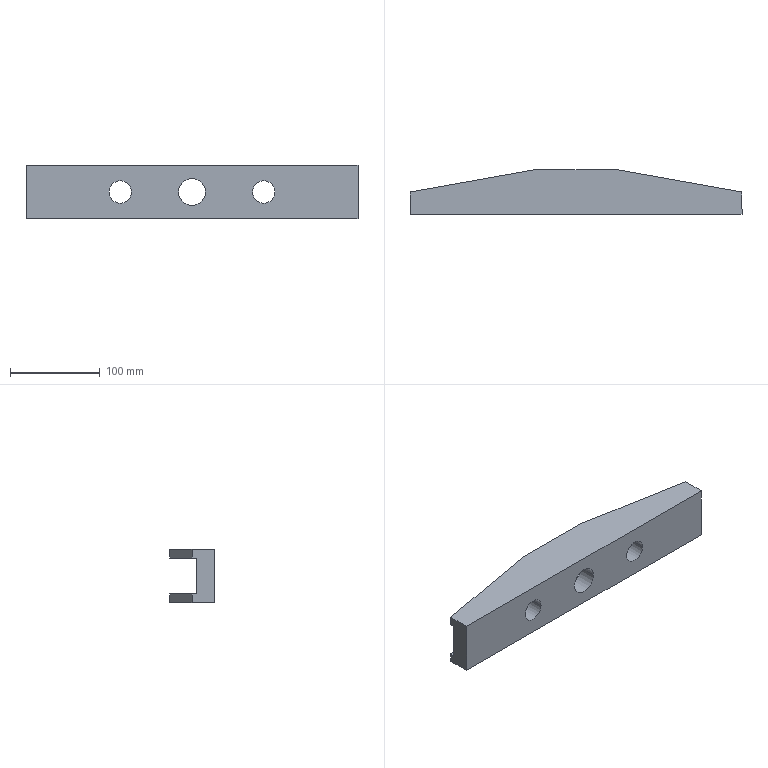Component | SolidWorks | SupportPlate-331-1 | 1 solid | 20 faces | box 370 x 50 x 60 mm | volume 562228 mm3 | plane 14 | cylinder 6 | commonest cylinder face diameters 25 x4 30 x2
build123d program:
from build123d import *

# Parameters (mm, degrees)
BOSS_EXTRUDE1_DEPTH = 60
SKETCH2_W           = 57.116
SKETCH2_H           = 40
CUT_EXTRUDE1_DEPTH  = 377.962
SKETCH3_R           = 15
SKETCH3_R_2         = 12.5
CUT_EXTRUDE2_DEPTH  = 197.787


with BuildPart() as part:
    # Sketch1 → Boss-Extrude1 (new body)
    with BuildSketch(Plane(origin=(0, 0, 0), x_dir=(1, 0, 0), z_dir=(0, 1, 0))):
        Polygon((-185, -15), (-45, 10), (45, 10), (185, -15), (185, -40), (-185, -40), align=None)
    extrude(amount=BOSS_EXTRUDE1_DEPTH)

    # Sketch2 → Cut-Extrude1 (cut, through all)
    with BuildSketch(Plane(origin=(185, 0, 0), x_dir=(0, 0, -1), z_dir=(1, 0, 0))):
        with Locations((8.558, 30)):
            Rectangle(SKETCH2_W, SKETCH2_H)
    extrude(amount=-CUT_EXTRUDE1_DEPTH, mode=Mode.SUBTRACT)

    # Sketch3 → Cut-Extrude2 (cut, through all)
    with BuildSketch(Plane(origin=(0, 0, 20), x_dir=(-1, 0, 0), z_dir=(0, 0, -1))):
        with Locations((0, 30)):
            Circle(SKETCH3_R)
        with Locations((-80, 30)):
            Circle(SKETCH3_R_2)
        with Locations((80, 30)):
            Circle(SKETCH3_R_2)
    extrude(amount=-CUT_EXTRUDE2_DEPTH, mode=Mode.SUBTRACT)


solid = part.part

# Placed as in the assembly
solid = solid.moved(Location((-101.681, 1325.897, 653.723), (90, 0, 0)))
STEP:
#1=COLOUR_RGB('',0.7922,0.8196,0.9333);
#2=FILL_AREA_STYLE_COLOUR('',#1);
#3=FILL_AREA_STYLE('',(#2));
#4=SURFACE_STYLE_FILL_AREA(#3);
#5=SURFACE_SIDE_STYLE('',(#4));
#6=SURFACE_STYLE_USAGE(.BOTH.,#5);
#7=PRESENTATION_STYLE_ASSIGNMENT((#6));
#8=CARTESIAN_POINT('',(-6.661,50.626,26.918));
#9=VERTEX_POINT('',#8);
#10=CARTESIAN_POINT('',(-7.645,50.626,26.918));
#11=VERTEX_POINT('',#10);
#12=CARTESIAN_POINT('',(-7.153,50.626,26.918));
#13=DIRECTION('',(-0.,1.,-0.));
#14=DIRECTION('',(-1.,0.,0.));
#15=AXIS2_PLACEMENT_3D('',#12,#13,#14);
#16=CIRCLE('',#15,0.4921);
#17=EDGE_CURVE('',#9,#11,#16,.T.);
#18=ORIENTED_EDGE('',*,*,#17,.F.);
#19=CARTESIAN_POINT('',(-6.661,51.413,26.918));
#20=VERTEX_POINT('',#19);
#21=CARTESIAN_POINT('',(-6.661,50.626,26.918));
#22=DIRECTION('',(-0.,1.,-0.));
#23=VECTOR('',#22,39.37);
#24=LINE('',#21,#23);
#25=EDGE_CURVE('',#9,#20,#24,.T.);
#26=ORIENTED_EDGE('',*,*,#25,.T.);
#27=CARTESIAN_POINT('',(-7.645,51.413,26.918));
#28=VERTEX_POINT('',#27);
#29=CARTESIAN_POINT('',(-7.153,51.413,26.918));
#30=DIRECTION('',(-0.,1.,-0.));
#31=DIRECTION('',(-1.,0.,0.));
#32=AXIS2_PLACEMENT_3D('',#29,#30,#31);
#33=CIRCLE('',#32,0.4921);
#34=EDGE_CURVE('',#20,#28,#33,.T.);
#35=ORIENTED_EDGE('',*,*,#34,.T.);
#36=CARTESIAN_POINT('',(-7.645,50.626,26.918));
#37=DIRECTION('',(-0.,1.,-0.));
#38=VECTOR('',#37,39.37);
#39=LINE('',#36,#38);
#40=EDGE_CURVE('',#11,#28,#39,.T.);
#41=ORIENTED_EDGE('',*,*,#40,.F.);
#42=EDGE_LOOP('',(#18,#26,#35,#41));
#43=FACE_OUTER_BOUND('',#42,.T.);
#44=CARTESIAN_POINT('',(-7.153,50.626,26.918));
#45=DIRECTION('',(-0.,1.,-0.));
#46=DIRECTION('',(-1.,0.,0.));
#47=AXIS2_PLACEMENT_3D('',#44,#45,#46);
#48=CYLINDRICAL_SURFACE('',#47,0.4921);
#49=ADVANCED_FACE('',(#43),#48,.F.);
#50=CARTESIAN_POINT('',(-0.3614,50.626,26.918));
#51=VERTEX_POINT('',#50);
#52=CARTESIAN_POINT('',(-1.346,50.626,26.918));
#53=VERTEX_POINT('',#52);
#54=CARTESIAN_POINT('',(-0.8536,50.626,26.918));
#55=DIRECTION('',(-0.,1.,-0.));
#56=DIRECTION('',(-1.,0.,0.));
#57=AXIS2_PLACEMENT_3D('',#54,#55,#56);
#58=CIRCLE('',#57,0.4921);
#59=EDGE_CURVE('',#51,#53,#58,.T.);
#60=ORIENTED_EDGE('',*,*,#59,.F.);
#61=CARTESIAN_POINT('',(-0.3614,51.413,26.918));
#62=VERTEX_POINT('',#61);
#63=CARTESIAN_POINT('',(-0.3614,50.626,26.918));
#64=DIRECTION('',(-0.,1.,-0.));
#65=VECTOR('',#64,39.37);
#66=LINE('',#63,#65);
#67=EDGE_CURVE('',#51,#62,#66,.T.);
#68=ORIENTED_EDGE('',*,*,#67,.T.);
#69=CARTESIAN_POINT('',(-1.346,51.413,26.918));
#70=VERTEX_POINT('',#69);
#71=CARTESIAN_POINT('',(-0.8536,51.413,26.918));
#72=DIRECTION('',(-0.,1.,-0.));
#73=DIRECTION('',(-1.,0.,0.));
#74=AXIS2_PLACEMENT_3D('',#71,#72,#73);
#75=CIRCLE('',#74,0.4921);
#76=EDGE_CURVE('',#62,#70,#75,.T.);
#77=ORIENTED_EDGE('',*,*,#76,.T.);
#78=CARTESIAN_POINT('',(-1.346,50.626,26.918));
#79=DIRECTION('',(-0.,1.,-0.));
#80=VECTOR('',#79,39.37);
#81=LINE('',#78,#80);
#82=EDGE_CURVE('',#53,#70,#81,.T.);
#83=ORIENTED_EDGE('',*,*,#82,.F.);
#84=EDGE_LOOP('',(#60,#68,#77,#83));
#85=FACE_OUTER_BOUND('',#84,.T.);
#86=CARTESIAN_POINT('',(-0.8536,50.626,26.918));
#87=DIRECTION('',(-0.,1.,-0.));
#88=DIRECTION('',(-1.,0.,0.));
#89=AXIS2_PLACEMENT_3D('',#86,#87,#88);
#90=CYLINDRICAL_SURFACE('',#89,0.4921);
#91=ADVANCED_FACE('',(#85),#90,.F.);
#92=CARTESIAN_POINT('',(-3.413,50.626,26.918));
#93=VERTEX_POINT('',#92);
#94=CARTESIAN_POINT('',(-4.594,50.626,26.918));
#95=VERTEX_POINT('',#94);
#96=CARTESIAN_POINT('',(-4.003,50.626,26.918));
#97=DIRECTION('',(-0.,1.,-0.));
#98=DIRECTION('',(-1.,0.,0.));
#99=AXIS2_PLACEMENT_3D('',#96,#97,#98);
#100=CIRCLE('',#99,0.5906);
#101=EDGE_CURVE('',#93,#95,#100,.T.);
#102=ORIENTED_EDGE('',*,*,#101,.F.);
#103=CARTESIAN_POINT('',(-3.413,51.413,26.918));
#104=VERTEX_POINT('',#103);
#105=CARTESIAN_POINT('',(-3.413,50.626,26.918));
#106=DIRECTION('',(-0.,1.,-0.));
#107=VECTOR('',#106,39.37);
#108=LINE('',#105,#107);
#109=EDGE_CURVE('',#93,#104,#108,.T.);
#110=ORIENTED_EDGE('',*,*,#109,.T.);
#111=CARTESIAN_POINT('',(-4.594,51.413,26.918));
#112=VERTEX_POINT('',#111);
#113=CARTESIAN_POINT('',(-4.003,51.413,26.918));
#114=DIRECTION('',(-0.,1.,-0.));
#115=DIRECTION('',(-1.,0.,0.));
#116=AXIS2_PLACEMENT_3D('',#113,#114,#115);
#117=CIRCLE('',#116,0.5906);
#118=EDGE_CURVE('',#104,#112,#117,.T.);
#119=ORIENTED_EDGE('',*,*,#118,.T.);
#120=CARTESIAN_POINT('',(-4.594,50.626,26.918));
#121=DIRECTION('',(-0.,1.,-0.));
#122=VECTOR('',#121,39.37);
#123=LINE('',#120,#122);
#124=EDGE_CURVE('',#95,#112,#123,.T.);
#125=ORIENTED_EDGE('',*,*,#124,.F.);
#126=EDGE_LOOP('',(#102,#110,#119,#125));
#127=FACE_OUTER_BOUND('',#126,.T.);
#128=CARTESIAN_POINT('',(-4.003,50.626,26.918));
#129=DIRECTION('',(-0.,1.,-0.));
#130=DIRECTION('',(-1.,0.,0.));
#131=AXIS2_PLACEMENT_3D('',#128,#129,#130);
#132=CYLINDRICAL_SURFACE('',#131,0.5906);
#133=ADVANCED_FACE('',(#127),#132,.F.);
#134=CARTESIAN_POINT('',(3.28,51.61,28.099));
#135=VERTEX_POINT('',#134);
#136=CARTESIAN_POINT('',(3.28,51.61,27.706));
#137=VERTEX_POINT('',#136);
#138=CARTESIAN_POINT('',(3.28,51.61,28.099));
#139=DIRECTION('',(-0.,-0.,-1.));
#140=VECTOR('',#139,39.37);
#141=LINE('',#138,#140);
#142=EDGE_CURVE('',#135,#137,#141,.T.);
#143=ORIENTED_EDGE('',*,*,#142,.T.);
#144=CARTESIAN_POINT('',(-2.232,52.594,27.706));
#145=VERTEX_POINT('',#144);
#146=CARTESIAN_POINT('',(3.28,51.61,27.706));
#147=DIRECTION('',(-0.9844,0.1758,0.));
#148=VECTOR('',#147,39.37);
#149=LINE('',#146,#148);
#150=EDGE_CURVE('',#137,#145,#149,.T.);
#151=ORIENTED_EDGE('',*,*,#150,.T.);
#152=CARTESIAN_POINT('',(-2.232,52.594,28.099));
#153=VERTEX_POINT('',#152);
#154=CARTESIAN_POINT('',(-2.232,52.594,28.099));
#155=DIRECTION('',(-0.,-0.,-1.));
#156=VECTOR('',#155,39.37);
#157=LINE('',#154,#156);
#158=EDGE_CURVE('',#153,#145,#157,.T.);
#159=ORIENTED_EDGE('',*,*,#158,.F.);
#160=CARTESIAN_POINT('',(3.28,51.61,28.099));
#161=DIRECTION('',(-0.9844,0.1758,0.));
#162=VECTOR('',#161,39.37);
#163=LINE('',#160,#162);
#164=EDGE_CURVE('',#135,#153,#163,.T.);
#165=ORIENTED_EDGE('',*,*,#164,.F.);
#166=EDGE_LOOP('',(#143,#151,#159,#165));
#167=FACE_OUTER_BOUND('',#166,.T.);
#168=CARTESIAN_POINT('',(3.28,51.61,28.099));
#169=DIRECTION('',(-0.1758,-0.9844,0.));
#170=DIRECTION('',(0.9844,-0.1758,-0.));
#171=AXIS2_PLACEMENT_3D('',#168,#169,#170);
#172=PLANE('',#171);
#173=ADVANCED_FACE('',(#167),#172,.F.);
#174=ORIENTED_EDGE('',*,*,#158,.T.);
#175=CARTESIAN_POINT('',(-5.775,52.594,27.706));
#176=VERTEX_POINT('',#175);
#177=CARTESIAN_POINT('',(-2.232,52.594,27.706));
#178=DIRECTION('',(-1.,-0.,0.));
#179=VECTOR('',#178,39.37);
#180=LINE('',#177,#179);
#181=EDGE_CURVE('',#145,#176,#180,.T.);
#182=ORIENTED_EDGE('',*,*,#181,.T.);
#183=CARTESIAN_POINT('',(-5.775,52.594,28.099));
#184=VERTEX_POINT('',#183);
#185=CARTESIAN_POINT('',(-5.775,52.594,28.099));
#186=DIRECTION('',(-0.,-0.,-1.));
#187=VECTOR('',#186,39.37);
#188=LINE('',#185,#187);
#189=EDGE_CURVE('',#184,#176,#188,.T.);
#190=ORIENTED_EDGE('',*,*,#189,.F.);
#191=CARTESIAN_POINT('',(-2.232,52.594,28.099));
#192=DIRECTION('',(-1.,-0.,0.));
#193=VECTOR('',#192,39.37);
#194=LINE('',#191,#193);
#195=EDGE_CURVE('',#153,#184,#194,.T.);
#196=ORIENTED_EDGE('',*,*,#195,.F.);
#197=EDGE_LOOP('',(#174,#182,#190,#196));
#198=FACE_OUTER_BOUND('',#197,.T.);
#199=CARTESIAN_POINT('',(-2.232,52.594,28.099));
#200=DIRECTION('',(0.,-1.,0.));
#201=DIRECTION('',(1.,0.,-0.));
#202=AXIS2_PLACEMENT_3D('',#199,#200,#201);
#203=PLANE('',#202);
#204=ADVANCED_FACE('',(#198),#203,.F.);
#205=ORIENTED_EDGE('',*,*,#189,.T.);
#206=CARTESIAN_POINT('',(-11.287,51.61,27.706));
#207=VERTEX_POINT('',#206);
#208=CARTESIAN_POINT('',(-11.287,51.61,27.706));
#209=DIRECTION('',(-0.9844,-0.1758,0.));
#210=VECTOR('',#209,39.37);
#211=LINE('',#208,#210);
#212=EDGE_CURVE('',#176,#207,#211,.T.);
#213=ORIENTED_EDGE('',*,*,#212,.T.);
#214=CARTESIAN_POINT('',(-11.287,51.61,28.099));
#215=VERTEX_POINT('',#214);
#216=CARTESIAN_POINT('',(-11.287,51.61,28.099));
#217=DIRECTION('',(-0.,-0.,-1.));
#218=VECTOR('',#217,39.37);
#219=LINE('',#216,#218);
#220=EDGE_CURVE('',#215,#207,#219,.T.);
#221=ORIENTED_EDGE('',*,*,#220,.F.);
#222=CARTESIAN_POINT('',(-11.287,51.61,28.099));
#223=DIRECTION('',(-0.9844,-0.1758,0.));
#224=VECTOR('',#223,39.37);
#225=LINE('',#222,#224);
#226=EDGE_CURVE('',#184,#215,#225,.T.);
#227=ORIENTED_EDGE('',*,*,#226,.F.);
#228=EDGE_LOOP('',(#205,#213,#221,#227));
#229=FACE_OUTER_BOUND('',#228,.T.);
#230=CARTESIAN_POINT('',(-11.287,51.61,28.099));
#231=DIRECTION('',(0.1758,-0.9844,0.));
#232=DIRECTION('',(0.9844,0.1758,-0.));
#233=AXIS2_PLACEMENT_3D('',#230,#231,#232);
#234=PLANE('',#233);
#235=ADVANCED_FACE('',(#229),#234,.F.);
#236=CARTESIAN_POINT('',(3.28,51.413,27.706));
#237=VERTEX_POINT('',#236);
#238=CARTESIAN_POINT('',(3.28,51.413,26.131));
#239=VERTEX_POINT('',#238);
#240=CARTESIAN_POINT('',(3.28,51.413,27.706));
#241=DIRECTION('',(-0.,-0.,-1.));
#242=VECTOR('',#241,39.37);
#243=LINE('',#240,#242);
#244=EDGE_CURVE('',#237,#239,#243,.T.);
#245=ORIENTED_EDGE('',*,*,#244,.F.);
#246=CARTESIAN_POINT('',(3.28,51.413,27.706));
#247=DIRECTION('',(-0.,-1.,0.));
#248=VECTOR('',#247,39.37);
#249=LINE('',#246,#248);
#250=EDGE_CURVE('',#137,#237,#249,.T.);
#251=ORIENTED_EDGE('',*,*,#250,.F.);
#252=ORIENTED_EDGE('',*,*,#142,.F.);
#253=CARTESIAN_POINT('',(3.28,50.626,28.099));
#254=VERTEX_POINT('',#253);
#255=CARTESIAN_POINT('',(3.28,50.626,28.099));
#256=DIRECTION('',(-0.,1.,-0.));
#257=VECTOR('',#256,39.37);
#258=LINE('',#255,#257);
#259=EDGE_CURVE('',#254,#135,#258,.T.);
#260=ORIENTED_EDGE('',*,*,#259,.F.);
#261=CARTESIAN_POINT('',(3.28,50.626,25.737));
#262=VERTEX_POINT('',#261);
#263=CARTESIAN_POINT('',(3.28,50.626,28.099));
#264=DIRECTION('',(-0.,-0.,-1.));
#265=VECTOR('',#264,39.37);
#266=LINE('',#263,#265);
#267=EDGE_CURVE('',#254,#262,#266,.T.);
#268=ORIENTED_EDGE('',*,*,#267,.T.);
#269=CARTESIAN_POINT('',(3.28,51.61,25.737));
#270=VERTEX_POINT('',#269);
#271=CARTESIAN_POINT('',(3.28,50.626,25.737));
#272=DIRECTION('',(-0.,1.,-0.));
#273=VECTOR('',#272,39.37);
#274=LINE('',#271,#273);
#275=EDGE_CURVE('',#262,#270,#274,.T.);
#276=ORIENTED_EDGE('',*,*,#275,.T.);
#277=CARTESIAN_POINT('',(3.28,51.61,26.131));
#278=VERTEX_POINT('',#277);
#279=CARTESIAN_POINT('',(3.28,51.61,28.099));
#280=DIRECTION('',(-0.,-0.,-1.));
#281=VECTOR('',#280,39.37);
#282=LINE('',#279,#281);
#283=EDGE_CURVE('',#278,#270,#282,.T.);
#284=ORIENTED_EDGE('',*,*,#283,.F.);
#285=CARTESIAN_POINT('',(3.28,51.413,26.131));
#286=DIRECTION('',(0.,1.,-0.));
#287=VECTOR('',#286,39.37);
#288=LINE('',#285,#287);
#289=EDGE_CURVE('',#239,#278,#288,.T.);
#290=ORIENTED_EDGE('',*,*,#289,.F.);
#291=EDGE_LOOP('',(#245,#251,#252,#260,#268,#276,#284,#290));
#292=FACE_OUTER_BOUND('',#291,.T.);
#293=CARTESIAN_POINT('',(3.28,50.626,28.099));
#294=DIRECTION('',(-1.,-0.,0.));
#295=DIRECTION('',(0.,-1.,0.));
#296=AXIS2_PLACEMENT_3D('',#293,#294,#295);
#297=PLANE('',#296);
#298=ADVANCED_FACE('',(#292),#297,.F.);
#299=CARTESIAN_POINT('',(-2.232,52.594,26.131));
#300=VERTEX_POINT('',#299);
#301=CARTESIAN_POINT('',(-2.232,52.594,25.737));
#302=VERTEX_POINT('',#301);
#303=CARTESIAN_POINT('',(-2.232,52.594,28.099));
#304=DIRECTION('',(-0.,-0.,-1.));
#305=VECTOR('',#304,39.37);
#306=LINE('',#303,#305);
#307=EDGE_CURVE('',#300,#302,#306,.T.);
#308=ORIENTED_EDGE('',*,*,#307,.F.);
#309=CARTESIAN_POINT('',(3.28,51.61,26.131));
#310=DIRECTION('',(0.9844,-0.1758,-0.));
#311=VECTOR('',#310,39.37);
#312=LINE('',#309,#311);
#313=EDGE_CURVE('',#300,#278,#312,.T.);
#314=ORIENTED_EDGE('',*,*,#313,.T.);
#315=ORIENTED_EDGE('',*,*,#283,.T.);
#316=CARTESIAN_POINT('',(3.28,51.61,25.737));
#317=DIRECTION('',(-0.9844,0.1758,0.));
#318=VECTOR('',#317,39.37);
#319=LINE('',#316,#318);
#320=EDGE_CURVE('',#270,#302,#319,.T.);
#321=ORIENTED_EDGE('',*,*,#320,.T.);
#322=EDGE_LOOP('',(#308,#314,#315,#321));
#323=FACE_OUTER_BOUND('',#322,.T.);
#324=CARTESIAN_POINT('',(3.28,51.61,28.099));
#325=DIRECTION('',(-0.1758,-0.9844,0.));
#326=DIRECTION('',(0.9844,-0.1758,-0.));
#327=AXIS2_PLACEMENT_3D('',#324,#325,#326);
#328=PLANE('',#327);
#329=ADVANCED_FACE('',(#323),#328,.F.);
#330=CARTESIAN_POINT('',(-5.775,52.594,26.131));
#331=VERTEX_POINT('',#330);
#332=CARTESIAN_POINT('',(-5.775,52.594,25.737));
#333=VERTEX_POINT('',#332);
#334=CARTESIAN_POINT('',(-5.775,52.594,28.099));
#335=DIRECTION('',(-0.,-0.,-1.));
#336=VECTOR('',#335,39.37);
#337=LINE('',#334,#336);
#338=EDGE_CURVE('',#331,#333,#337,.T.);
#339=ORIENTED_EDGE('',*,*,#338,.F.);
#340=CARTESIAN_POINT('',(-2.232,52.594,26.131));
#341=DIRECTION('',(1.,0.,-0.));
#342=VECTOR('',#341,39.37);
#343=LINE('',#340,#342);
#344=EDGE_CURVE('',#331,#300,#343,.T.);
#345=ORIENTED_EDGE('',*,*,#344,.T.);
#346=ORIENTED_EDGE('',*,*,#307,.T.);
#347=CARTESIAN_POINT('',(-2.232,52.594,25.737));
#348=DIRECTION('',(-1.,-0.,0.));
#349=VECTOR('',#348,39.37);
#350=LINE('',#347,#349);
#351=EDGE_CURVE('',#302,#333,#350,.T.);
#352=ORIENTED_EDGE('',*,*,#351,.T.);
#353=EDGE_LOOP('',(#339,#345,#346,#352));
#354=FACE_OUTER_BOUND('',#353,.T.);
#355=CARTESIAN_POINT('',(-2.232,52.594,28.099));
#356=DIRECTION('',(0.,-1.,0.));
#357=DIRECTION('',(1.,0.,-0.));
#358=AXIS2_PLACEMENT_3D('',#355,#356,#357);
#359=PLANE('',#358);
#360=ADVANCED_FACE('',(#354),#359,.F.);
#361=CARTESIAN_POINT('',(-11.287,51.61,26.131));
#362=VERTEX_POINT('',#361);
#363=CARTESIAN_POINT('',(-11.287,51.61,25.737));
#364=VERTEX_POINT('',#363);
#365=CARTESIAN_POINT('',(-11.287,51.61,28.099));
#366=DIRECTION('',(-0.,-0.,-1.));
#367=VECTOR('',#366,39.37);
#368=LINE('',#365,#367);
#369=EDGE_CURVE('',#362,#364,#368,.T.);
#370=ORIENTED_EDGE('',*,*,#369,.F.);
#371=CARTESIAN_POINT('',(-11.287,51.61,26.131));
#372=DIRECTION('',(0.9844,0.1758,-0.));
#373=VECTOR('',#372,39.37);
#374=LINE('',#371,#373);
#375=EDGE_CURVE('',#362,#331,#374,.T.);
#376=ORIENTED_EDGE('',*,*,#375,.T.);
#377=ORIENTED_EDGE('',*,*,#338,.T.);
#378=CARTESIAN_POINT('',(-11.287,51.61,25.737));
#379=DIRECTION('',(-0.9844,-0.1758,0.));
#380=VECTOR('',#379,39.37);
#381=LINE('',#378,#380);
#382=EDGE_CURVE('',#333,#364,#381,.T.);
#383=ORIENTED_EDGE('',*,*,#382,.T.);
#384=EDGE_LOOP('',(#370,#376,#377,#383));
#385=FACE_OUTER_BOUND('',#384,.T.);
#386=CARTESIAN_POINT('',(-11.287,51.61,28.099));
#387=DIRECTION('',(0.1758,-0.9844,0.));
#388=DIRECTION('',(0.9844,0.1758,-0.));
#389=AXIS2_PLACEMENT_3D('',#386,#387,#388);
#390=PLANE('',#389);
#391=ADVANCED_FACE('',(#385),#390,.F.);
#392=ORIENTED_EDGE('',*,*,#220,.T.);
#393=CARTESIAN_POINT('',(-11.287,51.413,27.706));
#394=VERTEX_POINT('',#393);
#395=CARTESIAN_POINT('',(-11.287,50.626,27.706));
#396=DIRECTION('',(0.,-1.,0.));
#397=VECTOR('',#396,39.37);
#398=LINE('',#395,#397);
#399=EDGE_CURVE('',#207,#394,#398,.T.);
#400=ORIENTED_EDGE('',*,*,#399,.T.);
#401=CARTESIAN_POINT('',(-11.287,51.413,26.131));
#402=VERTEX_POINT('',#401);
#403=CARTESIAN_POINT('',(-11.287,51.413,27.706));
#404=DIRECTION('',(-0.,-0.,-1.));
#405=VECTOR('',#404,39.37);
#406=LINE('',#403,#405);
#407=EDGE_CURVE('',#394,#402,#406,.T.);
#408=ORIENTED_EDGE('',*,*,#407,.T.);
#409=CARTESIAN_POINT('',(-11.287,51.413,26.131));
#410=DIRECTION('',(0.,1.,-0.));
#411=VECTOR('',#410,39.37);
#412=LINE('',#409,#411);
#413=EDGE_CURVE('',#402,#362,#412,.T.);
#414=ORIENTED_EDGE('',*,*,#413,.T.);
#415=ORIENTED_EDGE('',*,*,#369,.T.);
#416=CARTESIAN_POINT('',(-11.287,50.626,25.737));
#417=VERTEX_POINT('',#416);
#418=CARTESIAN_POINT('',(-11.287,50.626,25.737));
#419=DIRECTION('',(0.,-1.,0.));
#420=VECTOR('',#419,39.37);
#421=LINE('',#418,#420);
#422=EDGE_CURVE('',#364,#417,#421,.T.);
#423=ORIENTED_EDGE('',*,*,#422,.T.);
#424=CARTESIAN_POINT('',(-11.287,50.626,28.099));
#425=VERTEX_POINT('',#424);
#426=CARTESIAN_POINT('',(-11.287,50.626,28.099));
#427=DIRECTION('',(-0.,-0.,-1.));
#428=VECTOR('',#427,39.37);
#429=LINE('',#426,#428);
#430=EDGE_CURVE('',#425,#417,#429,.T.);
#431=ORIENTED_EDGE('',*,*,#430,.F.);
#432=CARTESIAN_POINT('',(-11.287,50.626,28.099));
#433=DIRECTION('',(0.,-1.,0.));
#434=VECTOR('',#433,39.37);
#435=LINE('',#432,#434);
#436=EDGE_CURVE('',#215,#425,#435,.T.);
#437=ORIENTED_EDGE('',*,*,#436,.F.);
#438=EDGE_LOOP('',(#392,#400,#408,#414,#415,#423,#431,#437));
#439=FACE_OUTER_BOUND('',#438,.T.);
#440=CARTESIAN_POINT('',(-11.287,50.626,28.099));
#441=DIRECTION('',(1.,0.,-0.));
#442=DIRECTION('',(-0.,1.,-0.));
#443=AXIS2_PLACEMENT_3D('',#440,#441,#442);
#444=PLANE('',#443);
#445=ADVANCED_FACE('',(#439),#444,.F.);
#446=CARTESIAN_POINT('',(-7.153,50.626,26.918));
#447=DIRECTION('',(-0.,1.,-0.));
#448=DIRECTION('',(-1.,0.,0.));
#449=AXIS2_PLACEMENT_3D('',#446,#447,#448);
#450=CIRCLE('',#449,0.4921);
#451=EDGE_CURVE('',#11,#9,#450,.T.);
#452=ORIENTED_EDGE('',*,*,#451,.T.);
#453=ORIENTED_EDGE('',*,*,#17,.T.);
#454=EDGE_LOOP('',(#452,#453));
#455=FACE_BOUND('',#454,.T.);
#456=CARTESIAN_POINT('',(-0.8536,50.626,26.918));
#457=DIRECTION('',(-0.,1.,-0.));
#458=DIRECTION('',(-1.,0.,0.));
#459=AXIS2_PLACEMENT_3D('',#456,#457,#458);
#460=CIRCLE('',#459,0.4921);
#461=EDGE_CURVE('',#53,#51,#460,.T.);
#462=ORIENTED_EDGE('',*,*,#461,.T.);
#463=ORIENTED_EDGE('',*,*,#59,.T.);
#464=EDGE_LOOP('',(#462,#463));
#465=FACE_BOUND('',#464,.T.);
#466=CARTESIAN_POINT('',(-4.003,50.626,26.918));
#467=DIRECTION('',(-0.,1.,-0.));
#468=DIRECTION('',(-1.,0.,0.));
#469=AXIS2_PLACEMENT_3D('',#466,#467,#468);
#470=CIRCLE('',#469,0.5906);
#471=EDGE_CURVE('',#95,#93,#470,.T.);
#472=ORIENTED_EDGE('',*,*,#471,.T.);
#473=ORIENTED_EDGE('',*,*,#101,.T.);
#474=EDGE_LOOP('',(#472,#473));
#475=FACE_BOUND('',#474,.T.);
#476=CARTESIAN_POINT('',(3.28,50.626,25.737));
#477=DIRECTION('',(1.,0.,-0.));
#478=VECTOR('',#477,39.37);
#479=LINE('',#476,#478);
#480=EDGE_CURVE('',#417,#262,#479,.T.);
#481=ORIENTED_EDGE('',*,*,#480,.T.);
#482=ORIENTED_EDGE('',*,*,#267,.F.);
#483=CARTESIAN_POINT('',(3.28,50.626,28.099));
#484=DIRECTION('',(1.,0.,-0.));
#485=VECTOR('',#484,39.37);
#486=LINE('',#483,#485);
#487=EDGE_CURVE('',#425,#254,#486,.T.);
#488=ORIENTED_EDGE('',*,*,#487,.F.);
#489=ORIENTED_EDGE('',*,*,#430,.T.);
#490=EDGE_LOOP('',(#481,#482,#488,#489));
#491=FACE_OUTER_BOUND('',#490,.T.);
#492=CARTESIAN_POINT('',(3.28,50.626,28.099));
#493=DIRECTION('',(-0.,1.,-0.));
#494=DIRECTION('',(-1.,-0.,0.));
#495=AXIS2_PLACEMENT_3D('',#492,#493,#494);
#496=PLANE('',#495);
#497=ADVANCED_FACE('',(#455,#465,#475,#491),#496,.F.);
#498=ORIENTED_EDGE('',*,*,#259,.T.);
#499=ORIENTED_EDGE('',*,*,#164,.T.);
#500=ORIENTED_EDGE('',*,*,#195,.T.);
#501=ORIENTED_EDGE('',*,*,#226,.T.);
#502=ORIENTED_EDGE('',*,*,#436,.T.);
#503=ORIENTED_EDGE('',*,*,#487,.T.);
#504=EDGE_LOOP('',(#498,#499,#500,#501,#502,#503));
#505=FACE_OUTER_BOUND('',#504,.T.);
#506=CARTESIAN_POINT('',(-4.003,52.201,28.099));
#507=DIRECTION('',(0.,0.,1.));
#508=DIRECTION('',(0.,-1.,0.));
#509=AXIS2_PLACEMENT_3D('',#506,#507,#508);
#510=PLANE('',#509);
#511=ADVANCED_FACE('',(#505),#510,.T.);
#512=ORIENTED_EDGE('',*,*,#275,.F.);
#513=ORIENTED_EDGE('',*,*,#480,.F.);
#514=ORIENTED_EDGE('',*,*,#422,.F.);
#515=ORIENTED_EDGE('',*,*,#382,.F.);
#516=ORIENTED_EDGE('',*,*,#351,.F.);
#517=ORIENTED_EDGE('',*,*,#320,.F.);
#518=EDGE_LOOP('',(#512,#513,#514,#515,#516,#517));
#519=FACE_OUTER_BOUND('',#518,.T.);
#520=CARTESIAN_POINT('',(-4.003,52.201,25.737));
#521=DIRECTION('',(0.,0.,1.));
#522=DIRECTION('',(0.,-1.,0.));
#523=AXIS2_PLACEMENT_3D('',#520,#521,#522);
#524=PLANE('',#523);
#525=ADVANCED_FACE('',(#519),#524,.F.);
#526=ORIENTED_EDGE('',*,*,#250,.T.);
#527=CARTESIAN_POINT('',(-11.287,51.413,27.706));
#528=DIRECTION('',(1.,0.,-0.));
#529=VECTOR('',#528,39.37);
#530=LINE('',#527,#529);
#531=EDGE_CURVE('',#394,#237,#530,.T.);
#532=ORIENTED_EDGE('',*,*,#531,.F.);
#533=ORIENTED_EDGE('',*,*,#399,.F.);
#534=ORIENTED_EDGE('',*,*,#212,.F.);
#535=ORIENTED_EDGE('',*,*,#181,.F.);
#536=ORIENTED_EDGE('',*,*,#150,.F.);
#537=EDGE_LOOP('',(#526,#532,#533,#534,#535,#536));
#538=FACE_OUTER_BOUND('',#537,.T.);
#539=CARTESIAN_POINT('',(-11.287,51.413,27.706));
#540=DIRECTION('',(0.,0.,1.));
#541=DIRECTION('',(0.,-1.,0.));
#542=AXIS2_PLACEMENT_3D('',#539,#540,#541);
#543=PLANE('',#542);
#544=ADVANCED_FACE('',(#538),#543,.F.);
#545=ORIENTED_EDGE('',*,*,#344,.F.);
#546=ORIENTED_EDGE('',*,*,#375,.F.);
#547=ORIENTED_EDGE('',*,*,#413,.F.);
#548=CARTESIAN_POINT('',(-11.287,51.413,26.131));
#549=DIRECTION('',(1.,0.,-0.));
#550=VECTOR('',#549,39.37);
#551=LINE('',#548,#550);
#552=EDGE_CURVE('',#402,#239,#551,.T.);
#553=ORIENTED_EDGE('',*,*,#552,.T.);
#554=ORIENTED_EDGE('',*,*,#289,.T.);
#555=ORIENTED_EDGE('',*,*,#313,.F.);
#556=EDGE_LOOP('',(#545,#546,#547,#553,#554,#555));
#557=FACE_OUTER_BOUND('',#556,.T.);
#558=CARTESIAN_POINT('',(-11.287,51.413,26.131));
#559=DIRECTION('',(-0.,-0.,-1.));
#560=DIRECTION('',(-0.,1.,-0.));
#561=AXIS2_PLACEMENT_3D('',#558,#559,#560);
#562=PLANE('',#561);
#563=ADVANCED_FACE('',(#557),#562,.F.);
#564=CARTESIAN_POINT('',(-7.153,51.413,26.918));
#565=DIRECTION('',(-0.,1.,-0.));
#566=DIRECTION('',(-1.,0.,0.));
#567=AXIS2_PLACEMENT_3D('',#564,#565,#566);
#568=CIRCLE('',#567,0.4921);
#569=EDGE_CURVE('',#28,#20,#568,.T.);
#570=ORIENTED_EDGE('',*,*,#569,.F.);
#571=ORIENTED_EDGE('',*,*,#34,.F.);
#572=EDGE_LOOP('',(#570,#571));
#573=FACE_BOUND('',#572,.T.);
#574=CARTESIAN_POINT('',(-0.8536,51.413,26.918));
#575=DIRECTION('',(-0.,1.,-0.));
#576=DIRECTION('',(-1.,0.,0.));
#577=AXIS2_PLACEMENT_3D('',#574,#575,#576);
#578=CIRCLE('',#577,0.4921);
#579=EDGE_CURVE('',#70,#62,#578,.T.);
#580=ORIENTED_EDGE('',*,*,#579,.F.);
#581=ORIENTED_EDGE('',*,*,#76,.F.);
#582=EDGE_LOOP('',(#580,#581));
#583=FACE_BOUND('',#582,.T.);
#584=CARTESIAN_POINT('',(-4.003,51.413,26.918));
#585=DIRECTION('',(-0.,1.,-0.));
#586=DIRECTION('',(-1.,0.,0.));
#587=AXIS2_PLACEMENT_3D('',#584,#585,#586);
#588=CIRCLE('',#587,0.5906);
#589=EDGE_CURVE('',#112,#104,#588,.T.);
#590=ORIENTED_EDGE('',*,*,#589,.F.);
#591=ORIENTED_EDGE('',*,*,#118,.F.);
#592=EDGE_LOOP('',(#590,#591));
#593=FACE_BOUND('',#592,.T.);
#594=ORIENTED_EDGE('',*,*,#244,.T.);
#595=ORIENTED_EDGE('',*,*,#552,.F.);
#596=ORIENTED_EDGE('',*,*,#407,.F.);
#597=ORIENTED_EDGE('',*,*,#531,.T.);
#598=EDGE_LOOP('',(#594,#595,#596,#597));
#599=FACE_OUTER_BOUND('',#598,.T.);
#600=CARTESIAN_POINT('',(-11.287,51.413,27.706));
#601=DIRECTION('',(0.,-1.,0.));
#602=DIRECTION('',(1.,0.,-0.));
#603=AXIS2_PLACEMENT_3D('',#600,#601,#602);
#604=PLANE('',#603);
#605=ADVANCED_FACE('',(#573,#583,#593,#599),#604,.F.);
#606=ORIENTED_EDGE('',*,*,#109,.F.);
#607=ORIENTED_EDGE('',*,*,#471,.F.);
#608=ORIENTED_EDGE('',*,*,#124,.T.);
#609=ORIENTED_EDGE('',*,*,#589,.T.);
#610=EDGE_LOOP('',(#606,#607,#608,#609));
#611=FACE_OUTER_BOUND('',#610,.T.);
#612=CARTESIAN_POINT('',(-4.003,50.626,26.918));
#613=DIRECTION('',(-0.,1.,-0.));
#614=DIRECTION('',(-1.,0.,0.));
#615=AXIS2_PLACEMENT_3D('',#612,#613,#614);
#616=CYLINDRICAL_SURFACE('',#615,0.5906);
#617=ADVANCED_FACE('',(#611),#616,.F.);
#618=ORIENTED_EDGE('',*,*,#67,.F.);
#619=ORIENTED_EDGE('',*,*,#461,.F.);
#620=ORIENTED_EDGE('',*,*,#82,.T.);
#621=ORIENTED_EDGE('',*,*,#579,.T.);
#622=EDGE_LOOP('',(#618,#619,#620,#621));
#623=FACE_OUTER_BOUND('',#622,.T.);
#624=CARTESIAN_POINT('',(-0.8536,50.626,26.918));
#625=DIRECTION('',(-0.,1.,-0.));
#626=DIRECTION('',(-1.,0.,0.));
#627=AXIS2_PLACEMENT_3D('',#624,#625,#626);
#628=CYLINDRICAL_SURFACE('',#627,0.4921);
#629=ADVANCED_FACE('',(#623),#628,.F.);
#630=ORIENTED_EDGE('',*,*,#25,.F.);
#631=ORIENTED_EDGE('',*,*,#451,.F.);
#632=ORIENTED_EDGE('',*,*,#40,.T.);
#633=ORIENTED_EDGE('',*,*,#569,.T.);
#634=EDGE_LOOP('',(#630,#631,#632,#633));
#635=FACE_OUTER_BOUND('',#634,.T.);
#636=CARTESIAN_POINT('',(-7.153,50.626,26.918));
#637=DIRECTION('',(-0.,1.,-0.));
#638=DIRECTION('',(-1.,0.,0.));
#639=AXIS2_PLACEMENT_3D('',#636,#637,#638);
#640=CYLINDRICAL_SURFACE('',#639,0.4921);
#641=ADVANCED_FACE('',(#635),#640,.F.);
#642=CLOSED_SHELL('',(#49,#91,#133,#173,#204,#235,#298,#329,#360,#391,#445,#497,#511,#525,#544,#563,#605,#617,#629,#641));
#643=MANIFOLD_SOLID_BREP('',#642);
#644=STYLED_ITEM('',(#7),#643);
#645=(LENGTH_UNIT()NAMED_UNIT(*)SI_UNIT($,.METRE.));
#646=LENGTH_MEASURE_WITH_UNIT(LENGTH_MEASURE(0.0254),#645);
#647=DIMENSIONAL_EXPONENTS(1.,0.,0.,0.,0.,0.,0.);
#648=(CONVERSION_BASED_UNIT('',#646)LENGTH_UNIT()NAMED_UNIT(#647));
#649=UNCERTAINTY_MEASURE_WITH_UNIT(LENGTH_MEASURE(0.00001),#648,'','');
#650=(NAMED_UNIT(*)PLANE_ANGLE_UNIT()SI_UNIT($,.RADIAN.));
#651=(NAMED_UNIT(*)SI_UNIT($,.STERADIAN.)SOLID_ANGLE_UNIT());
#652=(GEOMETRIC_REPRESENTATION_CONTEXT(3)GLOBAL_UNCERTAINTY_ASSIGNED_CONTEXT((#649))GLOBAL_UNIT_ASSIGNED_CONTEXT((#648,#650,#651))REPRESENTATION_CONTEXT('',''));
#653=MECHANICAL_DESIGN_GEOMETRIC_PRESENTATION_REPRESENTATION('',(#644),#652);
#654=PRESENTATION_LAYER_ASSIGNMENT('','',(#644));
#655=CARTESIAN_POINT('',(0.,0.,0.));
#656=DIRECTION('',(0.,0.,1.));
#657=DIRECTION('',(1.,0.,0.));
#658=AXIS2_PLACEMENT_3D('',#655,#656,#657);
#659=(LENGTH_UNIT()NAMED_UNIT(*)SI_UNIT($,.METRE.));
#660=LENGTH_MEASURE_WITH_UNIT(LENGTH_MEASURE(0.0254),#659);
#661=DIMENSIONAL_EXPONENTS(1.,0.,0.,0.,0.,0.,0.);
#662=(CONVERSION_BASED_UNIT('',#660)LENGTH_UNIT()NAMED_UNIT(#661));
#663=UNCERTAINTY_MEASURE_WITH_UNIT(LENGTH_MEASURE(0.00001),#662,'','');
#664=(NAMED_UNIT(*)PLANE_ANGLE_UNIT()SI_UNIT($,.RADIAN.));
#665=(NAMED_UNIT(*)SI_UNIT($,.STERADIAN.)SOLID_ANGLE_UNIT());
#666=(GEOMETRIC_REPRESENTATION_CONTEXT(3)GLOBAL_UNCERTAINTY_ASSIGNED_CONTEXT((#663))GLOBAL_UNIT_ASSIGNED_CONTEXT((#662,#664,#665))REPRESENTATION_CONTEXT('',''));
#667=ADVANCED_BREP_SHAPE_REPRESENTATION('',(#643,#658),#666);